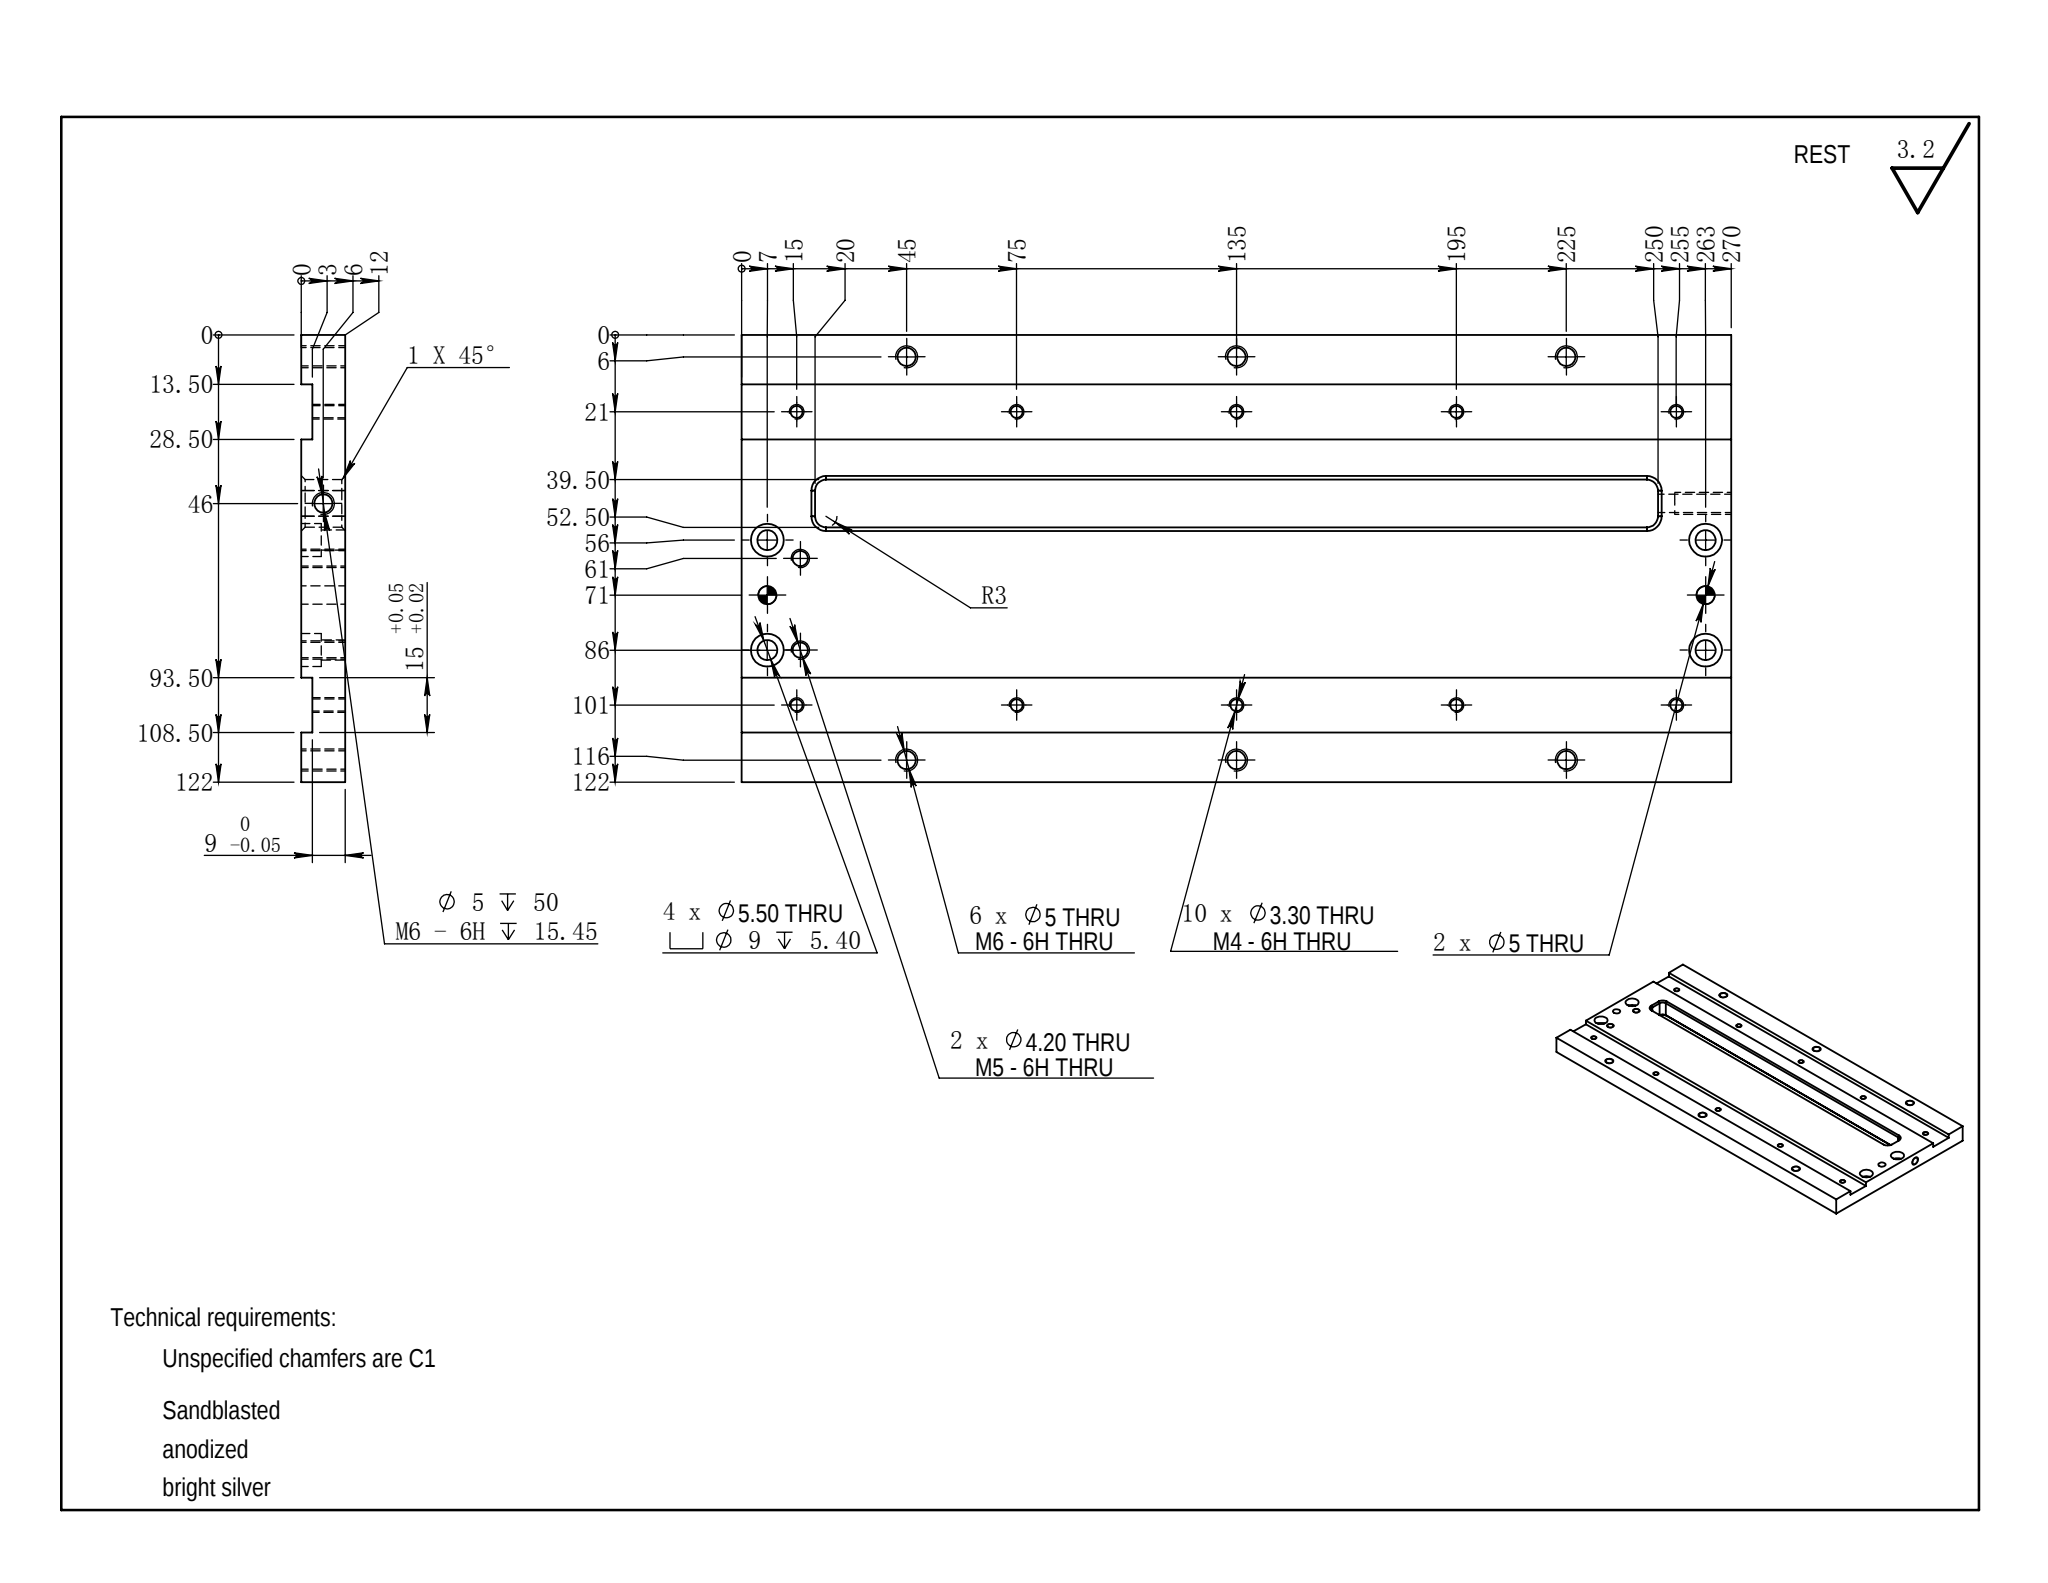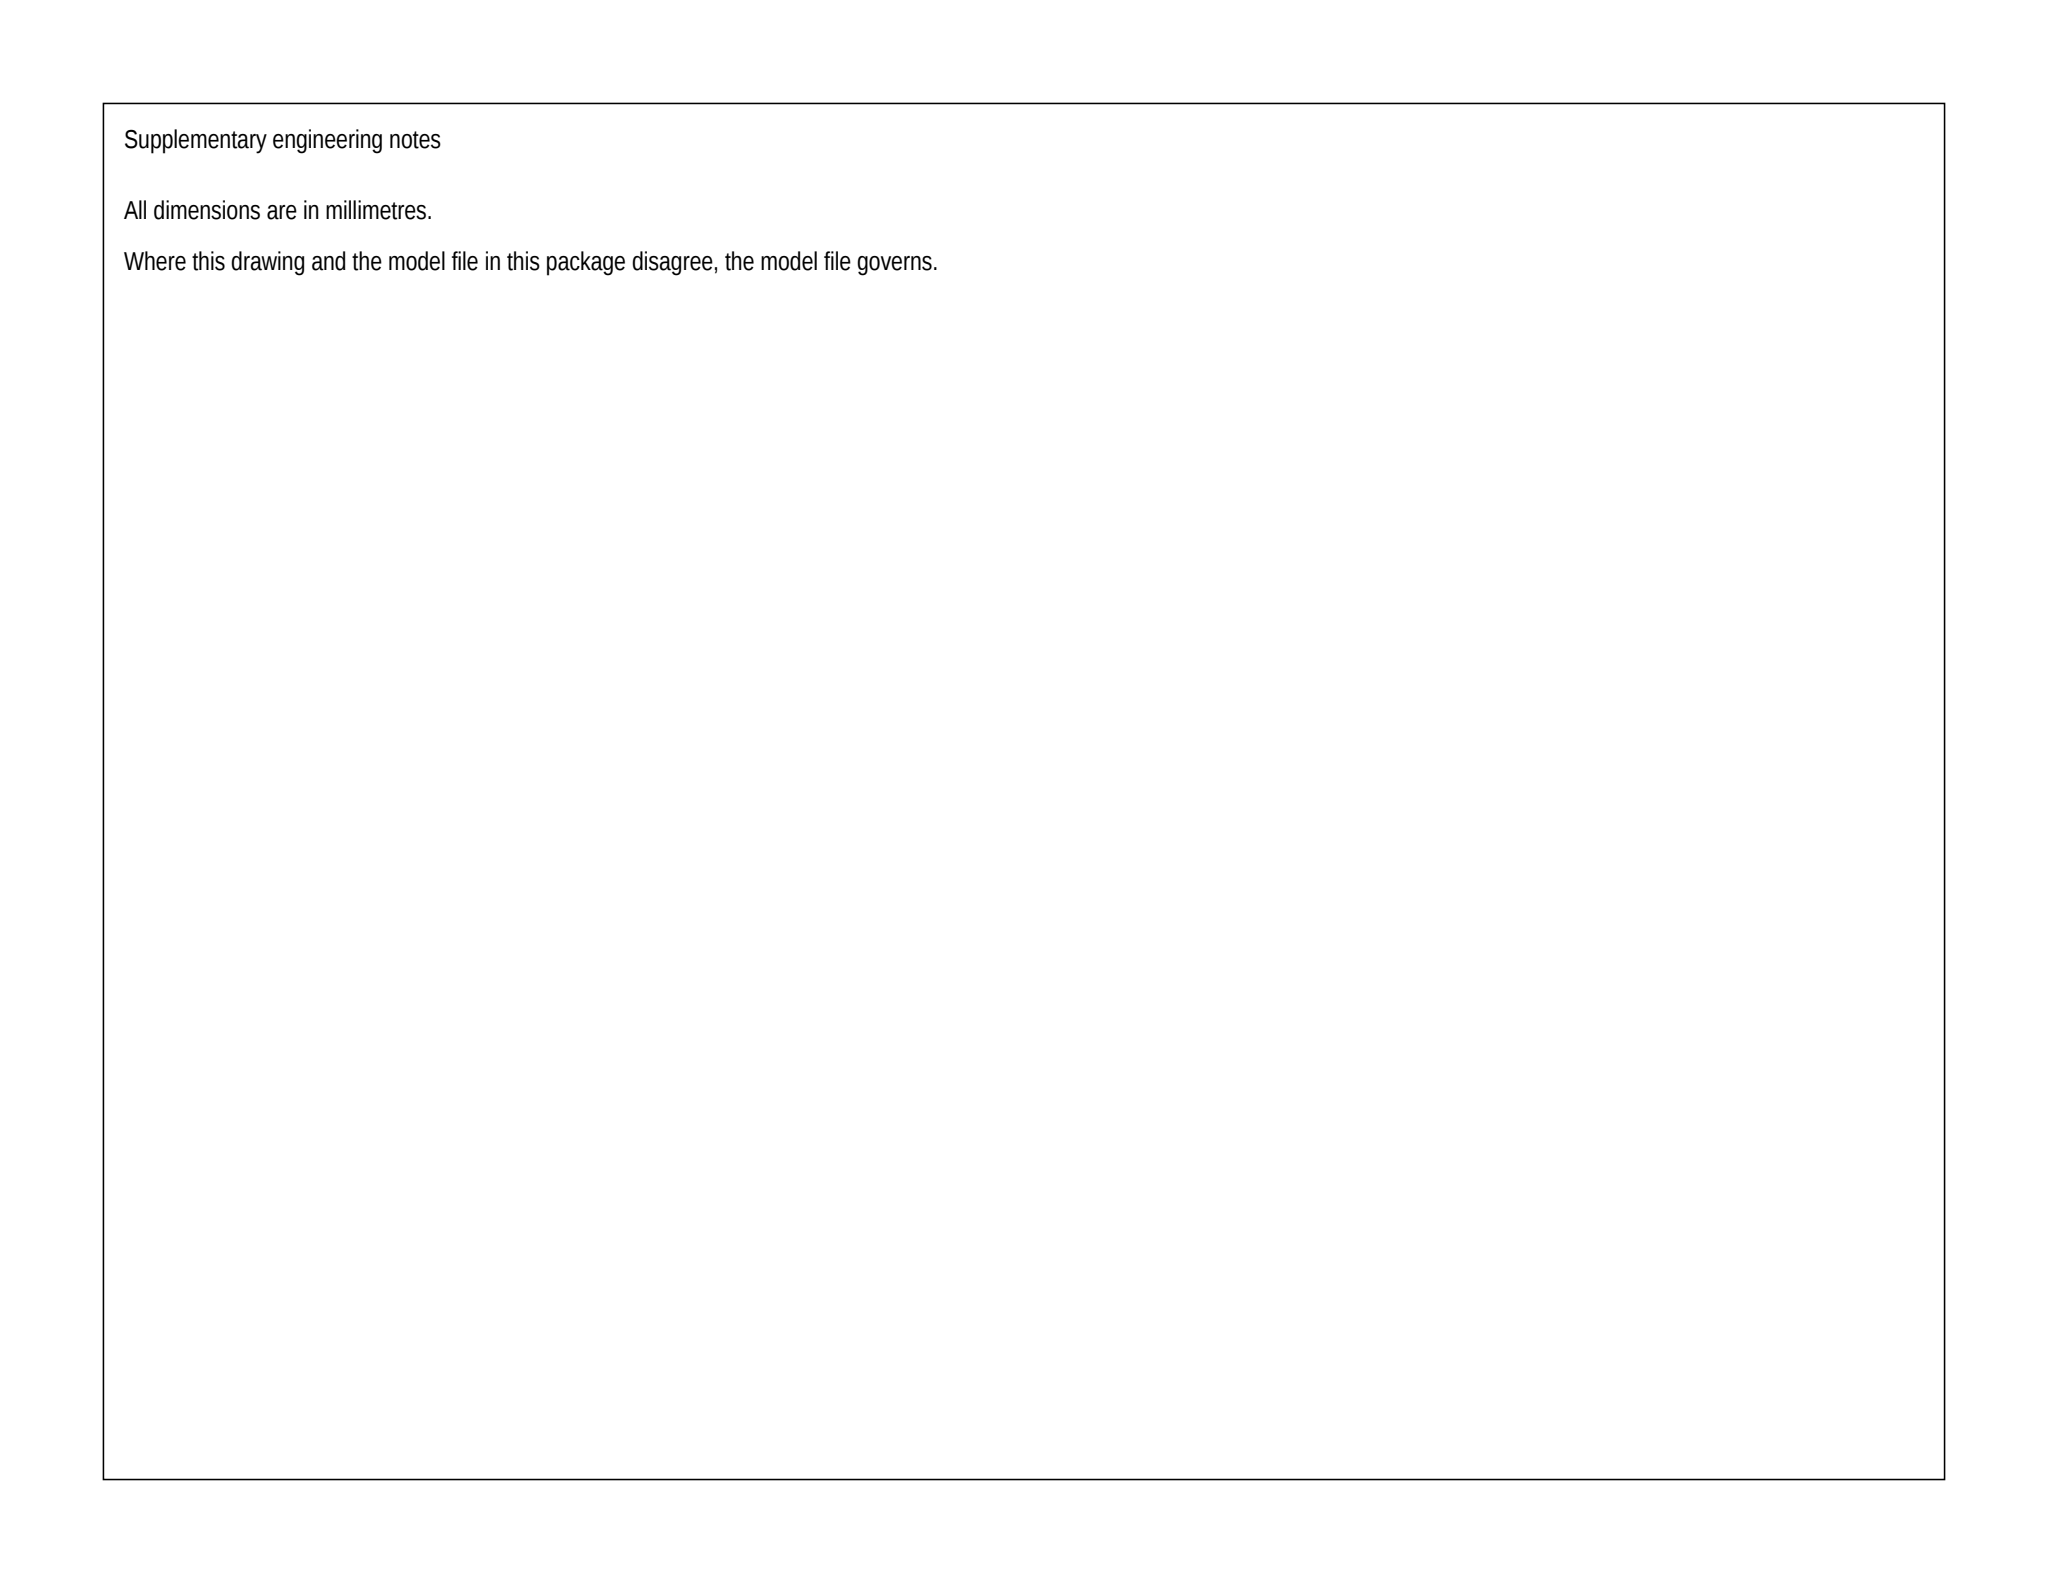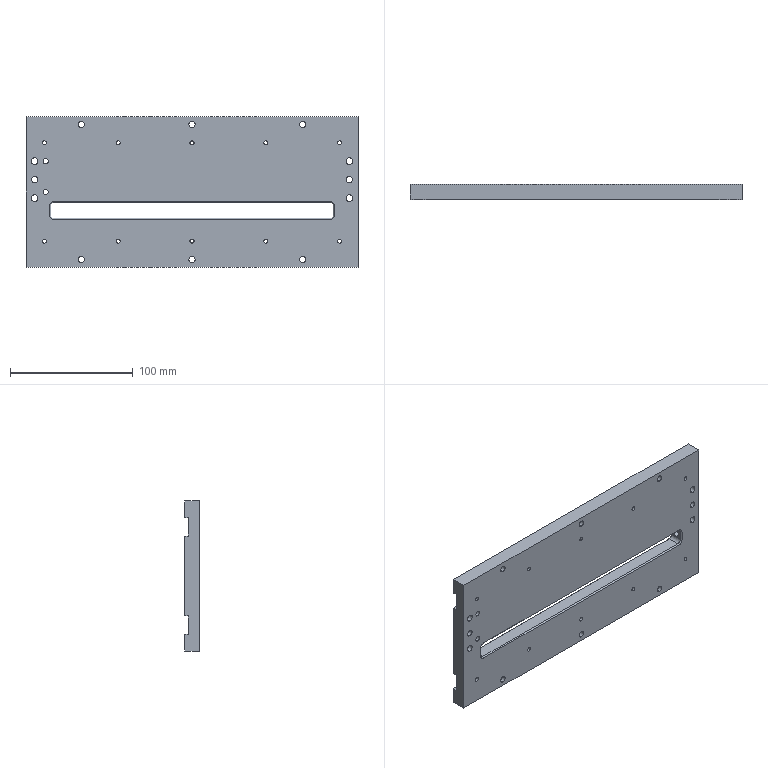Part | SolidWorks | mm | material A6061 | 1 solid | 100 faces | box 270 x 12 x 122 mm | volume 329328 mm3 | cylinder 62 | plane 30 | cone 8 | commonest cylinder face diameters 3.3 x20 5 x18 9 x8 5.5 x8 4.2 x4 6 x4
Drawing notes:
2X Ø4.2 (M5-6H) THRU AT X=16 FROM LEFT EDGE, Z=61 & 86 | from the solid: hole/bore dia 4.2, axis y, at [16,-,61] and [16,-,86], from 0 to 12 (full 12 thk)
10X M4-6H THRU, Ø3.3 TAP DRILL | from the solid: 10 holes dia 3.3 axis y at x=15,75,135,195,255 and z=21 & 101, from 0 to 9
2X M5-6H THRU, Ø4.2 TAP DRILL | from the solid: 2 holes dia 4.2 axis y at [16,-,61],[16,-,86], thru 12 thk
4X Ø5.5 THRU, C'BORE Ø9 DEPTH 5.4 FROM Y=12 FACE; AT X=7 AND X=263, Z=56 AND Z=86 (FROM MIN CORNER DATUM) | from the solid: cylinders: Ø5.5 axis y at (7,56),(7,86),(263,56),(263,86) from y=0 to 6.6; Ø9 axis y same positions from y=6.6 to 12.0
6X Ø5 THRU (12 THICK); AT X=45, 135, 225 ON Z=6 AND Z=116 | from the solid: cylinders: Ø5.0 axis y at (45,6),(135,6),(225,6),(45,116),(135,116),(225,116) from y=0 to 12.0
2X Ø5 THRU (12 THICK) AT X=7 AND X=263, Z=71 | from the solid: cylinders: Ø5.0 axis y at (7,71) and (263,71) from y=0 to 12.0
1X Ø5 CROSS HOLE IN X=270 END FACE, AXIS AT Y=6 AND Z=46, DEPTH 20 (X=270 TO X=250, BREAKS INTO SLOT) | from the solid: cylinders: Ø5.0 axis x at (y=6, z=46) from x=250.0 to x=270.0
SLOT IS THROUGH THE FULL 12 PLATE THICKNESS: 13 WIDE (Z=39.5 TO 52.5) X 230 LONG (X=20 TO 250), R3 CORNERS, 1X45° CHAMFER BOTH FACES | from the solid: axis_planes z=39.5 and z=52.5 extent y[1,11]; end planes x=20 and x=250 extent y[1,11] z[42.5,49.5]; concave arcs Ø6 y from 1 to 11; inclined planes 45° at y=0-1 and y=11-12 along slot edges
10X Ø3.3 (M4-6H) HOLES BREAK OUT AT THE 9 DEEP STEP FACE: DRILL DEPTH 9 FROM Y=0 (Z=21 AND Z=101 ROWS) | from the solid: cylinders: Ø3.3 axis y at z=21 and z=101 rows from y=0.0 to y=9.0; axis_planes y=9.0 at z[13.5,28.5] and z[93.5,108.5]
ALL DIMENSIONS IN MILLIMETRES | from the solid: STEP model facts given in mm; bbox_xyz = 270.0 x 12.0 x 122.0 mm
build123d program:
from build123d import *

# Parameters (mm, degrees)
SKETCH1_W                                       = 270
SKETCH1_H                                       = 122
BOSS_EXTRUDE1_DEPTH                             = 12
SKETCH2_W                                       = 270
SKETCH2_H                                       = 15
CUT_EXTRUDE1_DEPTH                              = 3
SKETCH3_W                                       = 230
SKETCH3_H                                       = 13
CUT_EXTRUDE2_DEPTH                              = 149.627
M5_HEX_SOCKET_HEAD_CAP_SCREW_CBORE1_D           = 5.5
M5_HEX_SOCKET_HEAD_CAP_SCREW_CBORE1_CBORE_D     = 9
M5_HEX_SOCKET_HEAD_CAP_SCREW_CBORE1_CBORE_DEPTH = 5.4
F_5_0_5_DIAMETER_HOLE1_D                        = 5
FILLET1_R                                       = 3
CHAMFER1_SIZE                                   = 1
M6_TAPPED_HOLE1_D                               = 5
M6_TAPPED_HOLE1_DEPTH                           = 50
M6_TAPPED_HOLE1_TIP                             = 1.502
M4_TAPPED_HOLE1_D                               = 3.3
LPATTERN1_COUNT                                 = 5
LPATTERN1_PITCH                                 = 60
M6_TAPPED_HOLE2_D                               = 5
M5_TAPPED_HOLE1_D                               = 4.2


with BuildPart() as part:
    # Sketch1 → Boss-Extrude1 (new body)
    with BuildSketch(Plane(origin=(0, 0, 0), x_dir=(1, 0, 0), z_dir=(0, 1, 0))):
        Rectangle(SKETCH1_W, SKETCH1_H)
    extrude(amount=BOSS_EXTRUDE1_DEPTH)

    # Sketch2 → Cut-Extrude1 (cut)
    with BuildSketch(Plane(origin=(0, 12, 0), x_dir=(1, 0, 0), z_dir=(0, 1, 0))):
        with Locations((0, 40)):
            Rectangle(SKETCH2_W, SKETCH2_H)
        with Locations((0, -40)):
            Rectangle(SKETCH2_W, SKETCH2_H)
    extrude(amount=-CUT_EXTRUDE1_DEPTH, mode=Mode.SUBTRACT)

    # Sketch3 → Cut-Extrude2 (cut, through all)
    with BuildSketch(Plane(origin=(0, 12, 0), x_dir=(1, 0, 0), z_dir=(0, 1, 0))):
        with Locations((0, 15)):
            Rectangle(SKETCH3_W, SKETCH3_H)
    extrude(amount=-CUT_EXTRUDE2_DEPTH, mode=Mode.SUBTRACT)

    # M5 Hex Socket Head Cap Screw CBORE1 (through all)
    with Locations(Plane(origin=(0, 12, 0), x_dir=(1, 0, 0), z_dir=(0, 1, 0))):
        with Locations((128, -25), (128, 5)):
            m5_hex_socket_head_cap_screw_cbore1 = CounterBoreHole(M5_HEX_SOCKET_HEAD_CAP_SCREW_CBORE1_D / 2, M5_HEX_SOCKET_HEAD_CAP_SCREW_CBORE1_CBORE_D / 2, M5_HEX_SOCKET_HEAD_CAP_SCREW_CBORE1_CBORE_DEPTH)

    # 5.0 _5_ Diameter Hole1 (through all)
    with Locations(Plane(origin=(0, 12, 0), x_dir=(1, 0, 0), z_dir=(0, 1, 0))):
        with Locations((128, -10)):
            f_5_0_5_diameter_hole1 = Hole(F_5_0_5_DIAMETER_HOLE1_D / 2)

    # Mirror1: M5 Hex Socket Head Cap Screw CBORE1, 5.0 _5_ Diameter Hole1 across plane
    add(m5_hex_socket_head_cap_screw_cbore1.mirror(Plane(origin=(0, 0, 0), x_dir=(0, 0, 1), z_dir=(1, 0, 0))), mode=Mode.SUBTRACT)
    add(f_5_0_5_diameter_hole1.mirror(Plane(origin=(0, 0, 0), x_dir=(0, 0, 1), z_dir=(1, 0, 0))), mode=Mode.SUBTRACT)

    # Fillet1
    fillet1_edges = [part.edges().sort_by_distance(p)[0] for p in [
        (115, 6, -21.5),
        (115, 6, -8.5),
        (-115, 6, -8.5),
        (-115, 6, -21.5),
    ]]
    fillet(fillet1_edges, radius=FILLET1_R)

    # Chamfer1
    chamfer1_edges = [part.edges().sort_by_distance(p)[0] for p in [
        (115, 12, -15),
        (115, 0, -15),
        (0, 12, -8.5),
        (0, 0, -8.5),
        (0, 12, -21.5),
        (0, 0, -21.5),
        (-115, 12, -15),
        (-115, 0, -15),
        (114.121, 12, -9.379),
        (114.121, 0, -9.379),
        (114.121, 12, -20.621),
        (114.121, 0, -20.621),
        (-114.121, 12, -9.379),
        (-114.121, 0, -9.379),
        (-114.121, 12, -20.621),
        (-114.121, 0, -20.621),
    ]]
    chamfer(chamfer1_edges, length=CHAMFER1_SIZE)

    # M6 Tapped Hole1
    with Locations(Plane(origin=(135, 0, 0), x_dir=(0, 0, -1), z_dir=(1, 0, 0))):
        with Locations((15, 6)):
            Hole(M6_TAPPED_HOLE1_D / 2, depth=M6_TAPPED_HOLE1_DEPTH)
            with Locations((0, 0, -(M6_TAPPED_HOLE1_DEPTH + M6_TAPPED_HOLE1_TIP / 2))):  # 118° drill point
                Cone(0, M6_TAPPED_HOLE1_D / 2, M6_TAPPED_HOLE1_TIP, mode=Mode.SUBTRACT)

    # M4 Tapped Hole1 (through all)
    with Locations(Plane(origin=(0, 9, 0), x_dir=(1, 0, 0), z_dir=(0, 1, 0))):
        with Locations((120, 40), (120, -40)):
            m4_tapped_hole1 = Hole(M4_TAPPED_HOLE1_D / 2)

    # LPattern1: M4 Tapped Hole1 ×5
    with Locations(*[(-i * LPATTERN1_PITCH, 0, 0) for i in range(1, LPATTERN1_COUNT)]):
        add(m4_tapped_hole1, mode=Mode.SUBTRACT)

    # M6 Tapped Hole2 (through all)
    with Locations(Plane(origin=(0, 12, 0), x_dir=(1, 0, 0), z_dir=(0, 1, 0))):
        with Locations((-90, 55), (0, 55), (90, 55), (-90, -55), (0, -55), (90, -55)):
            Hole(M6_TAPPED_HOLE2_D / 2)

    # M5 Tapped Hole1 (through all)
    with Locations(Plane(origin=(0, 12, 0), x_dir=(1, 0, 0), z_dir=(0, 1, 0))):
        with Locations((-119, 0), (-119, -25)):
            Hole(M5_TAPPED_HOLE1_D / 2)


solid = part.part